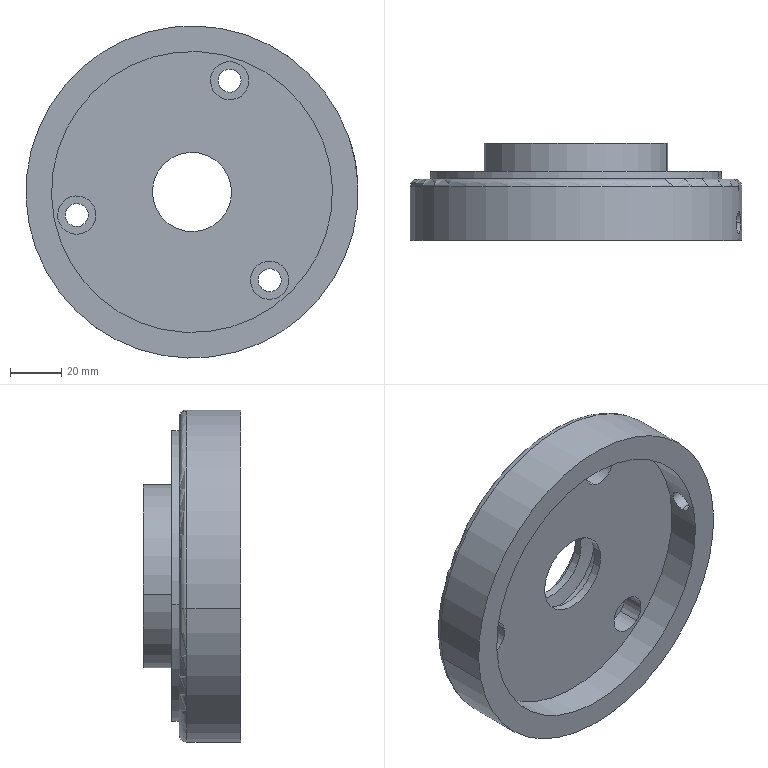Component | SolidWorks | 9-1 | 1 solid | 47 faces | box 130 x 38 x 130 mm | volume 216865 mm3 | cylinder 30 | plane 9 | torus 4 | cone 4 | commonest cylinder face diameters 15 x6 9 x6 31 x4 8.5 x2 44 x2 60 x2 110 x2 72 x2
build123d program:
from build123d import *

# Parameters (mm, degrees)
SKETCH1_R              = 65
BOSS_EXTRUDE1_DEPTH    = 24
SKETCH2_R              = 36
BOSS_EXTRUDE2_DEPTH    = 14
SKETCH4_R              = 57
BOSS_EXTRUDE3_DEPTH    = 3
SKETCH5_R              = 55
CUT_EXTRUDE1_DEPTH     = 13
SKETCH6_R              = 30
CUT_EXTRUDE2_DEPTH     = 11
HOLE1_D                = 9
HOLE1_DEPTH            = 99.955
HOLE1_CBORE_D          = 15
HOLE1_CBORE_DEPTH      = 9
CIRPATTERN1_COUNT      = 3
FILLET1_R              = 3
FILLET2_R              = 3
M10_TAPPED_HOLE2_D     = 8.5
M10_TAPPED_HOLE2_DEPTH = 24.5
M10_TAPPED_HOLE2_TIP   = 2.554


with BuildPart() as part:
    # Sketch1 → Boss-Extrude1 (new body)
    with BuildSketch(Plane(origin=(0, 0, 0), x_dir=(1, 0, 0), z_dir=(0, 1, 0))):
        with Locations(Location((0, 0, 0), (0, 0, 270))):
            Circle(SKETCH1_R)
    extrude(amount=BOSS_EXTRUDE1_DEPTH)

    # Sketch2 → Boss-Extrude2 (add)
    with BuildSketch(Plane(origin=(0, 24, 0), x_dir=(1, 0, 0), z_dir=(0, 1, 0))):
        with Locations(Location((0, 0, 0), (0, 0, 270))):
            Circle(SKETCH2_R)
    extrude(amount=BOSS_EXTRUDE2_DEPTH)

    # Sketch4 → Boss-Extrude3 (add)
    with BuildSketch(Plane(origin=(0, 24, 0), x_dir=(1, 0, 0), z_dir=(0, 1, 0))):
        with Locations(Location((0, 0, 0), (0, 0, 270))):
            Circle(SKETCH4_R)
    extrude(amount=BOSS_EXTRUDE3_DEPTH)

    # Sketch5 → Cut-Extrude1 (cut)
    with BuildSketch(Plane.XZ):
        with Locations(Location((0, 0, 0), (0, 0, 270))):
            Circle(SKETCH5_R)
    extrude(amount=-CUT_EXTRUDE1_DEPTH, mode=Mode.SUBTRACT)

    # Sketch6 → Cut-Extrude2 (cut)
    with BuildSketch(Plane(origin=(0, 38, 0), x_dir=(1, 0, 0), z_dir=(0, 1, 0))):
        with Locations(Location((0, 0, 0), (0, 0, 270))):
            Circle(SKETCH6_R)
    extrude(amount=-CUT_EXTRUDE2_DEPTH, mode=Mode.SUBTRACT)

    # Sketch8 → Cut-Revolve1 (revolve, cut)
    with BuildSketch(Plane(origin=(0, 0, 0), x_dir=(0, 0, -1), z_dir=(1, 0, 0))):
        Polygon((0, 0), (-15.5, 0), (-15.5, 16.202), (-22, 17), (-22, 23), (-15.5, 23.798), (-15.5, 27), (0, 27), align=None)
    revolve(axis=Axis((0, 27, 0), (0, -1, 0)), mode=Mode.SUBTRACT)

    # Hole1
    with Locations(Plane(origin=(0, 13, 0), x_dir=(-1, 0, 0), z_dir=(0, -1, 0))):
        with Locations((0, -46)):
            hole1 = CounterBoreHole(HOLE1_D / 2, HOLE1_CBORE_D / 2, HOLE1_CBORE_DEPTH, depth=HOLE1_DEPTH)

    # CirPattern1: Hole1 ×3 about axis
    cirpattern1_axis = Axis((0, 0, 0), (0, 1, 0))
    for i in range(1, CIRPATTERN1_COUNT):
        add(hole1.rotate(cirpattern1_axis, i * 360 / CIRPATTERN1_COUNT), mode=Mode.SUBTRACT)

    # Fillet1
    fillet1_edges = [part.edges().sort_by_distance(p)[0] for p in [
        (0, 27, -30),
    ]]
    fillet(fillet1_edges, radius=FILLET1_R)

    # Fillet2
    fillet2_edges = [part.edges().sort_by_distance(p)[0] for p in [
        (0, 24, -65),
    ]]
    fillet(fillet2_edges, radius=FILLET2_R)

    # M10 Tapped Hole2
    with Locations(Plane(origin=(0, 7, -65), x_dir=(1, 0, 0), z_dir=(0, 0, -1))):
        with Locations((0, 0)):
            Hole(M10_TAPPED_HOLE2_D / 2, depth=M10_TAPPED_HOLE2_DEPTH)
            with Locations((0, 0, -(M10_TAPPED_HOLE2_DEPTH + M10_TAPPED_HOLE2_TIP / 2))):  # 118° drill point
                Cone(0, M10_TAPPED_HOLE2_D / 2, M10_TAPPED_HOLE2_TIP, mode=Mode.SUBTRACT)


solid = part.part

# Placed as in the assembly
solid = solid.moved(Location((0, -326.2, 0), (-180, -78.666, 180)))